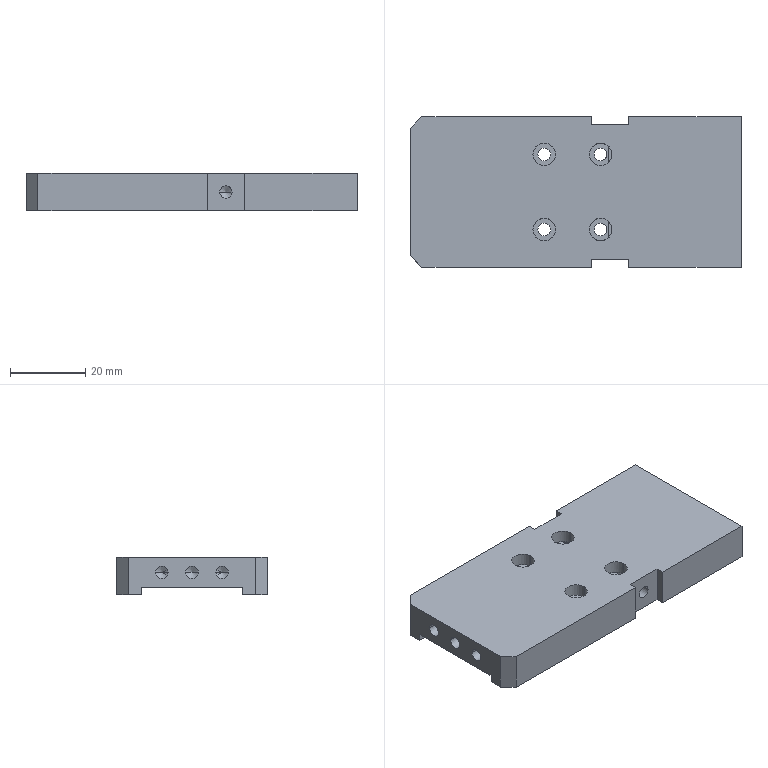Component | SolidWorks | 09HHHHH3-1 | 1 solid | 70 faces | box 88 x 40 x 10 mm | volume 28789 mm3 | cylinder 30 | plane 26 | cone 14 | commonest cylinder face diameters 3.3 x14 6 x8 3.4 x8
build123d program:
from build123d import *

# Parameters (mm, degrees)
SKETCH1_W                                            = 40
SKETCH1_H                                            = 10
BOSS_EXTRUDE1_DEPTH                                  = 88
SKETCH2_W                                            = 27
SKETCH2_H                                            = 2
CUT_EXTRUDE1_DEPTH                                   = 334.103
M4_TAPPED_HOLE1_D                                    = 3.3
M4_TAPPED_HOLE1_DEPTH                                = 10.1
M4_TAPPED_HOLE1_TIP                                  = 0.9914
M4_TAPPED_HOLE2_D                                    = 3.3
M4_TAPPED_HOLE2_DEPTH                                = 10.1
M4_TAPPED_HOLE2_TIP                                  = 0.9914
CHAMFER1_SIZE                                        = 3
HOLE_SIZE_ACCORDING_TO_THE_TYPE_OF_HEXAG_D           = 3.4
HOLE_SIZE_ACCORDING_TO_THE_TYPE_OF_HEXAG_CBORE_D     = 6
HOLE_SIZE_ACCORDING_TO_THE_TYPE_OF_HEXAG_CBORE_DEPTH = 3.4
SKETCH9_W                                            = 2
SKETCH9_H                                            = 10
CUT_EXTRUDE2_DEPTH                                   = 334.159
M4_TAPPED_HOLE3_D                                    = 3.3
M4_TAPPED_HOLE3_DEPTH                                = 10.1
M4_TAPPED_HOLE3_TIP                                  = 0.9914
M4_TAPPED_HOLE4_D                                    = 3.3
M4_TAPPED_HOLE4_DEPTH                                = 10.1
M4_TAPPED_HOLE4_TIP                                  = 0.9914


with BuildPart() as part:
    # Sketch1 → Boss-Extrude1 (new body)
    with BuildSketch(Plane.XY):
        with Locations((301.171, -2.921)):
            Rectangle(SKETCH1_W, SKETCH1_H)
    extrude(amount=BOSS_EXTRUDE1_DEPTH)

    # Sketch2 → Cut-Extrude1 (cut, through all)
    with BuildSketch(Plane.XY.offset(88)):
        with Locations((301.171, -6.921)):
            Rectangle(SKETCH2_W, SKETCH2_H)
    extrude(amount=-CUT_EXTRUDE1_DEPTH, mode=Mode.SUBTRACT)

    # M4 Tapped Hole1
    with Locations(Plane(origin=(0, 0, 0), x_dir=(-1, 0, 0), z_dir=(0, 0, -1))):
        with Locations((-311.171, -2.921), (-291.171, -2.921)):
            Hole(M4_TAPPED_HOLE1_D / 2, depth=M4_TAPPED_HOLE1_DEPTH)
            with Locations((0, 0, -(M4_TAPPED_HOLE1_DEPTH + M4_TAPPED_HOLE1_TIP / 2))):  # 118° drill point
                Cone(0, M4_TAPPED_HOLE1_D / 2, M4_TAPPED_HOLE1_TIP, mode=Mode.SUBTRACT)

    # M4 Tapped Hole2
    with Locations(Plane.XY.offset(88)):
        with Locations((293.171, -1.921), (301.171, -1.921), (309.171, -1.921)):
            Hole(M4_TAPPED_HOLE2_D / 2, depth=M4_TAPPED_HOLE2_DEPTH)
            with Locations((0, 0, -(M4_TAPPED_HOLE2_DEPTH + M4_TAPPED_HOLE2_TIP / 2))):  # 118° drill point
                Cone(0, M4_TAPPED_HOLE2_D / 2, M4_TAPPED_HOLE2_TIP, mode=Mode.SUBTRACT)

    # Chamfer1
    chamfer1_edges = [part.edges().sort_by_distance(p)[0] for p in [
        (321.171, -2.921, 88),
        (281.171, -2.921, 88),
    ]]
    chamfer(chamfer1_edges, length=CHAMFER1_SIZE)

    # Hole Size according to the type of hexag (through all)
    with Locations(Plane(origin=(0, 2.079, 0), x_dir=(1, 0, 0), z_dir=(0, 1, 0))):
        with Locations((311.171, -37.45), (311.171, -52.45), (291.171, -37.45), (291.171, -52.45)):
            CounterBoreHole(HOLE_SIZE_ACCORDING_TO_THE_TYPE_OF_HEXAG_D / 2, HOLE_SIZE_ACCORDING_TO_THE_TYPE_OF_HEXAG_CBORE_D / 2, HOLE_SIZE_ACCORDING_TO_THE_TYPE_OF_HEXAG_CBORE_DEPTH)

    # Sketch9 → Cut-Extrude2 (cut, through all)
    with BuildSketch(Plane(origin=(0, 2.079, 0), x_dir=(1, 0, 0), z_dir=(0, 1, 0))):
        with Locations((282.171, -35)):
            Rectangle(SKETCH9_W, SKETCH9_H)
        with Locations((320.171, -35)):
            Rectangle(SKETCH9_W, SKETCH9_H)
    extrude(amount=-CUT_EXTRUDE2_DEPTH, mode=Mode.SUBTRACT)

    # M4 Tapped Hole3
    with Locations(Plane.ZY.offset(-283.171)):
        with Locations((35, -2.921)):
            Hole(M4_TAPPED_HOLE3_D / 2, depth=M4_TAPPED_HOLE3_DEPTH)
            with Locations((0, 0, -(M4_TAPPED_HOLE3_DEPTH + M4_TAPPED_HOLE3_TIP / 2))):  # 118° drill point
                Cone(0, M4_TAPPED_HOLE3_D / 2, M4_TAPPED_HOLE3_TIP, mode=Mode.SUBTRACT)

    # M4 Tapped Hole4
    with Locations(Plane(origin=(319.171, 0, 0), x_dir=(0, 0, -1), z_dir=(1, 0, 0))):
        with Locations((-35, -2.921)):
            Hole(M4_TAPPED_HOLE4_D / 2, depth=M4_TAPPED_HOLE4_DEPTH)
            with Locations((0, 0, -(M4_TAPPED_HOLE4_DEPTH + M4_TAPPED_HOLE4_TIP / 2))):  # 118° drill point
                Cone(0, M4_TAPPED_HOLE4_D / 2, M4_TAPPED_HOLE4_TIP, mode=Mode.SUBTRACT)


solid = part.part

# Placed as in the assembly
solid = solid.moved(Location((-562.94, 14.788, 6.765), (90, -90, 0)))